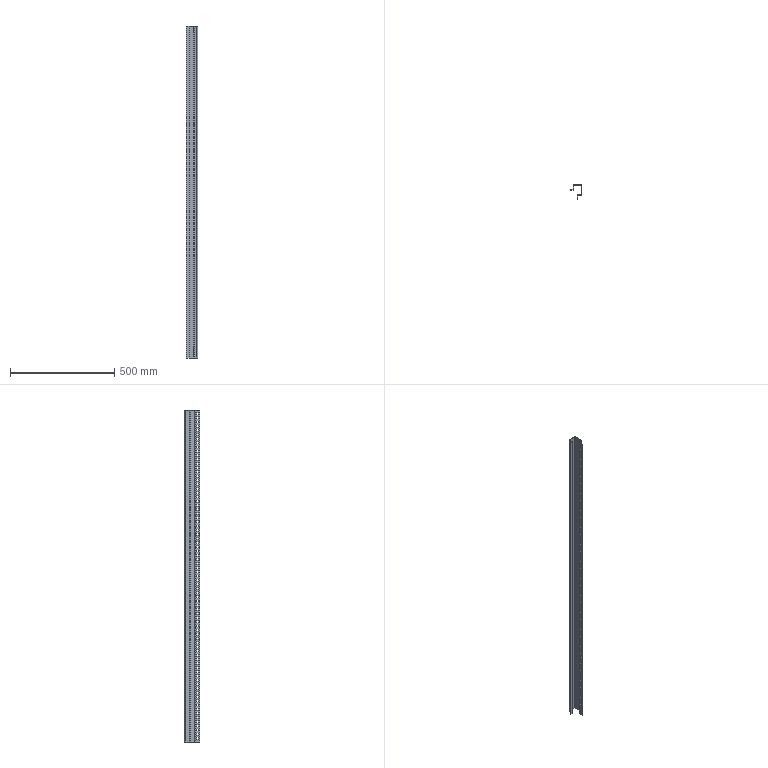Component | SolidWorks | Column-4 | 1 solid | 362 faces | volume 509430 mm3 | plane 352 | cylinder 10 | commonest cylinder face diameters 6 x5 2 x5